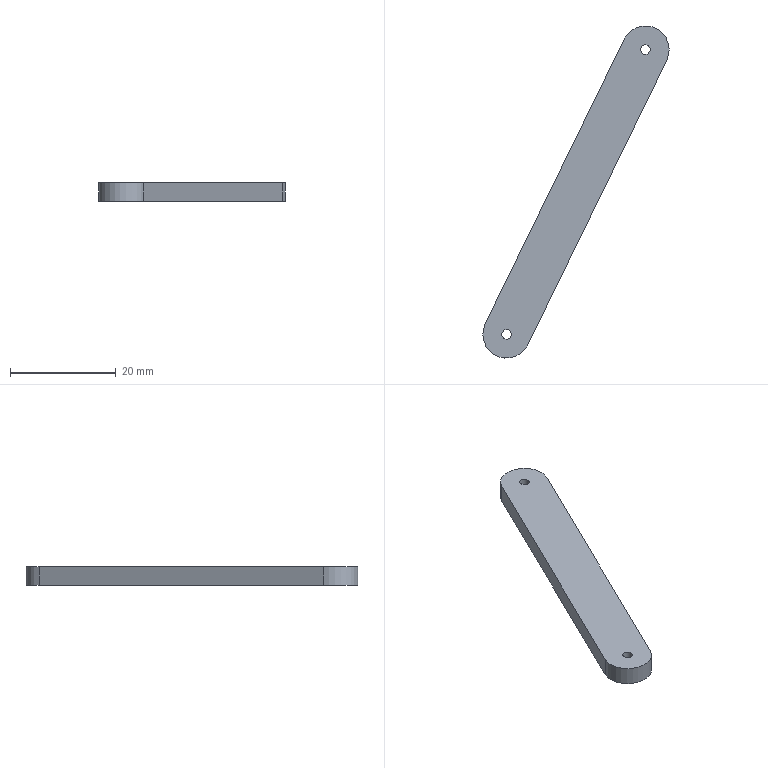Component | NX | SPEAKER_MOUNT | 1 solid | 8 faces | box 35.3 x 62.93 x 3.5 mm | volume 2095 mm3 | cylinder 4 | plane 4 | commonest cylinder face diameters 9 x2 1.8 x2
STEP:
#1=CARTESIAN_POINT('',(0.,0.,0.));
#2=DIRECTION('',(0.,0.,1.));
#3=DIRECTION('',(1.,0.,0.));
#4=AXIS2_PLACEMENT_3D('',#1,#2,#3);
#5=CARTESIAN_POINT('',(33.172,-30.052,31.776));
#6=VERTEX_POINT('',#5);
#7=CARTESIAN_POINT('',(33.172,-30.052,28.276));
#8=VERTEX_POINT('',#7);
#9=CARTESIAN_POINT('',(33.172,-30.052,31.776));
#10=DIRECTION('',(0.,0.,-1.));
#11=VECTOR('',#10,1.);
#12=LINE('',#9,#11);
#13=CARTESIAN_POINT('',(29.127,-28.08,31.776));
#14=DIRECTION('',(0.,0.,-1.));
#15=DIRECTION('',(-1.,0.,0.));
#16=AXIS2_PLACEMENT_3D('',#13,#14,#15);
#17=CYLINDRICAL_SURFACE('',#16,4.5);
#18=CARTESIAN_POINT('',(3.595,0.));
#19=DIRECTION('',(0.,1.));
#20=VECTOR('',#19,1.);
#21=LINE('',#18,#20);
#22=(GEOMETRIC_REPRESENTATION_CONTEXT(2)PARAMETRIC_REPRESENTATION_CONTEXT()REPRESENTATION_CONTEXT('',''));
#23=DEFINITIONAL_REPRESENTATION('',(#21),#22);
#24=PCURVE('',#17,#23);
#25=CARTESIAN_POINT('',(33.172,-30.052,31.776));
#26=DIRECTION('',(-0.8988,0.4384,0.));
#27=DIRECTION('',(-0.4384,-0.8988,0.));
#28=AXIS2_PLACEMENT_3D('',#25,#26,#27);
#29=PLANE('',#28);
#30=CARTESIAN_POINT('',(0.,0.));
#31=DIRECTION('',(0.,-1.));
#32=VECTOR('',#31,1.);
#33=LINE('',#30,#32);
#34=(GEOMETRIC_REPRESENTATION_CONTEXT(2)PARAMETRIC_REPRESENTATION_CONTEXT()REPRESENTATION_CONTEXT('',''));
#35=DEFINITIONAL_REPRESENTATION('',(#33),#34);
#36=PCURVE('',#29,#35);
#37=SURFACE_CURVE('',#12,(#24,#36),.PCURVE_S1.);
#38=EDGE_CURVE('',#6,#8,#37,.T.);
#39=ORIENTED_EDGE('',*,*,#38,.F.);
#40=CARTESIAN_POINT('',(25.083,-26.107,31.776));
#41=VERTEX_POINT('',#40);
#42=CARTESIAN_POINT('',(29.127,-28.08,31.776));
#43=DIRECTION('',(0.,0.,-1.));
#44=DIRECTION('',(1.,0.,0.));
#45=AXIS2_PLACEMENT_3D('',#42,#43,#44);
#46=CIRCLE('',#45,4.5);
#47=CARTESIAN_POINT('',(3.142,0.));
#48=DIRECTION('',(1.,0.));
#49=VECTOR('',#48,1.);
#50=LINE('',#47,#49);
#51=(GEOMETRIC_REPRESENTATION_CONTEXT(2)PARAMETRIC_REPRESENTATION_CONTEXT()REPRESENTATION_CONTEXT('',''));
#52=DEFINITIONAL_REPRESENTATION('',(#50),#51);
#53=PCURVE('',#17,#52);
#54=CARTESIAN_POINT('',(29.127,-28.08,31.776));
#55=DIRECTION('',(0.,0.,1.));
#56=DIRECTION('',(1.,0.,0.));
#57=AXIS2_PLACEMENT_3D('',#54,#55,#56);
#58=PLANE('',#57);
#59=CARTESIAN_POINT('',(4.5,-0.));
#60=CARTESIAN_POINT('',(4.5,-7.794));
#61=CARTESIAN_POINT('',(-2.25,-3.897));
#62=CARTESIAN_POINT('',(-9.,-0.));
#63=CARTESIAN_POINT('',(-2.25,3.897));
#64=CARTESIAN_POINT('',(4.5,7.794));
#65=CARTESIAN_POINT('',(4.5,-0.));
#66=(BOUNDED_CURVE()B_SPLINE_CURVE(2,(#59,#60,#61,#62,#63,#64,#65),.UNSPECIFIED.,.T.,.F.)B_SPLINE_CURVE_WITH_KNOTS((1,2,2,2,2,1),(-2.094,0.,2.094,4.189,6.283,8.378),.UNSPECIFIED.)CURVE()GEOMETRIC_REPRESENTATION_ITEM()RATIONAL_B_SPLINE_CURVE((1.,0.5,1.,0.5,1.,0.5,1.))REPRESENTATION_ITEM(''));
#67=(GEOMETRIC_REPRESENTATION_CONTEXT(2)PARAMETRIC_REPRESENTATION_CONTEXT()REPRESENTATION_CONTEXT('',''));
#68=DEFINITIONAL_REPRESENTATION('',(#66),#67);
#69=PCURVE('',#58,#68);
#70=SURFACE_CURVE('',#46,(#53,#69),.PCURVE_S1.);
#71=EDGE_CURVE('',#6,#41,#70,.T.);
#72=ORIENTED_EDGE('',*,*,#71,.T.);
#73=CARTESIAN_POINT('',(25.083,-26.107,28.276));
#74=VERTEX_POINT('',#73);
#75=CARTESIAN_POINT('',(25.083,-26.107,31.776));
#76=DIRECTION('',(0.,0.,-1.));
#77=VECTOR('',#76,1.);
#78=LINE('',#75,#77);
#79=CARTESIAN_POINT('',(6.737,0.));
#80=DIRECTION('',(0.,1.));
#81=VECTOR('',#80,1.);
#82=LINE('',#79,#81);
#83=(GEOMETRIC_REPRESENTATION_CONTEXT(2)PARAMETRIC_REPRESENTATION_CONTEXT()REPRESENTATION_CONTEXT('',''));
#84=DEFINITIONAL_REPRESENTATION('',(#82),#83);
#85=PCURVE('',#17,#84);
#86=CARTESIAN_POINT('',(51.385,27.821,31.776));
#87=DIRECTION('',(0.8988,-0.4384,0.));
#88=DIRECTION('',(0.4384,0.8988,0.));
#89=AXIS2_PLACEMENT_3D('',#86,#87,#88);
#90=PLANE('',#89);
#91=CARTESIAN_POINT('',(-60.,0.));
#92=DIRECTION('',(0.,-1.));
#93=VECTOR('',#92,1.);
#94=LINE('',#91,#93);
#95=(GEOMETRIC_REPRESENTATION_CONTEXT(2)PARAMETRIC_REPRESENTATION_CONTEXT()REPRESENTATION_CONTEXT('',''));
#96=DEFINITIONAL_REPRESENTATION('',(#94),#95);
#97=PCURVE('',#90,#96);
#98=SURFACE_CURVE('',#78,(#85,#97),.PCURVE_S1.);
#99=EDGE_CURVE('',#41,#74,#98,.T.);
#100=ORIENTED_EDGE('',*,*,#99,.T.);
#101=CARTESIAN_POINT('',(29.127,-28.08,28.276));
#102=DIRECTION('',(0.,0.,-1.));
#103=DIRECTION('',(1.,0.,0.));
#104=AXIS2_PLACEMENT_3D('',#101,#102,#103);
#105=CIRCLE('',#104,4.5);
#106=CARTESIAN_POINT('',(3.142,3.5));
#107=DIRECTION('',(1.,0.));
#108=VECTOR('',#107,1.);
#109=LINE('',#106,#108);
#110=(GEOMETRIC_REPRESENTATION_CONTEXT(2)PARAMETRIC_REPRESENTATION_CONTEXT()REPRESENTATION_CONTEXT('',''));
#111=DEFINITIONAL_REPRESENTATION('',(#109),#110);
#112=PCURVE('',#17,#111);
#113=CARTESIAN_POINT('',(29.127,-28.08,28.276));
#114=DIRECTION('',(0.,0.,1.));
#115=DIRECTION('',(1.,0.,0.));
#116=AXIS2_PLACEMENT_3D('',#113,#114,#115);
#117=PLANE('',#116);
#118=CARTESIAN_POINT('',(4.5,-0.));
#119=CARTESIAN_POINT('',(4.5,-7.794));
#120=CARTESIAN_POINT('',(-2.25,-3.897));
#121=CARTESIAN_POINT('',(-9.,-0.));
#122=CARTESIAN_POINT('',(-2.25,3.897));
#123=CARTESIAN_POINT('',(4.5,7.794));
#124=CARTESIAN_POINT('',(4.5,-0.));
#125=(BOUNDED_CURVE()B_SPLINE_CURVE(2,(#118,#119,#120,#121,#122,#123,#124),.UNSPECIFIED.,.T.,.F.)B_SPLINE_CURVE_WITH_KNOTS((1,2,2,2,2,1),(-2.094,0.,2.094,4.189,6.283,8.378),.UNSPECIFIED.)CURVE()GEOMETRIC_REPRESENTATION_ITEM()RATIONAL_B_SPLINE_CURVE((1.,0.5,1.,0.5,1.,0.5,1.))REPRESENTATION_ITEM(''));
#126=(GEOMETRIC_REPRESENTATION_CONTEXT(2)PARAMETRIC_REPRESENTATION_CONTEXT()REPRESENTATION_CONTEXT('',''));
#127=DEFINITIONAL_REPRESENTATION('',(#125),#126);
#128=PCURVE('',#117,#127);
#129=SURFACE_CURVE('',#105,(#112,#128),.PCURVE_S1.);
#130=EDGE_CURVE('',#8,#74,#129,.T.);
#131=ORIENTED_EDGE('',*,*,#130,.F.);
#132=EDGE_LOOP('',(#39,#72,#100,#131));
#133=FACE_BOUND('',#132,.T.);
#134=ADVANCED_FACE('',(#133),#17,.T.);
#135=CARTESIAN_POINT('',(30.027,-28.08,31.776));
#136=VERTEX_POINT('',#135);
#137=CARTESIAN_POINT('',(29.127,-28.08,31.776));
#138=DIRECTION('',(0.,0.,-1.));
#139=DIRECTION('',(1.,0.,0.));
#140=AXIS2_PLACEMENT_3D('',#137,#138,#139);
#141=CIRCLE('',#140,0.9);
#142=CARTESIAN_POINT('',(29.127,-28.08,31.776));
#143=DIRECTION('',(0.,0.,-1.));
#144=DIRECTION('',(-1.,0.,0.));
#145=AXIS2_PLACEMENT_3D('',#142,#143,#144);
#146=CYLINDRICAL_SURFACE('',#145,0.9);
#147=CARTESIAN_POINT('',(3.142,0.));
#148=DIRECTION('',(1.,0.));
#149=VECTOR('',#148,1.);
#150=LINE('',#147,#149);
#151=(GEOMETRIC_REPRESENTATION_CONTEXT(2)PARAMETRIC_REPRESENTATION_CONTEXT()REPRESENTATION_CONTEXT('',''));
#152=DEFINITIONAL_REPRESENTATION('',(#150),#151);
#153=PCURVE('',#146,#152);
#154=CARTESIAN_POINT('',(0.9,0.));
#155=CARTESIAN_POINT('',(0.9,-1.559));
#156=CARTESIAN_POINT('',(-0.45,-0.7794));
#157=CARTESIAN_POINT('',(-1.8,-0.));
#158=CARTESIAN_POINT('',(-0.45,0.7794));
#159=CARTESIAN_POINT('',(0.9,1.559));
#160=CARTESIAN_POINT('',(0.9,0.));
#161=(BOUNDED_CURVE()B_SPLINE_CURVE(2,(#154,#155,#156,#157,#158,#159,#160),.UNSPECIFIED.,.T.,.F.)B_SPLINE_CURVE_WITH_KNOTS((1,2,2,2,2,1),(-2.094,0.,2.094,4.189,6.283,8.378),.UNSPECIFIED.)CURVE()GEOMETRIC_REPRESENTATION_ITEM()RATIONAL_B_SPLINE_CURVE((1.,0.5,1.,0.5,1.,0.5,1.))REPRESENTATION_ITEM(''));
#162=(GEOMETRIC_REPRESENTATION_CONTEXT(2)PARAMETRIC_REPRESENTATION_CONTEXT()REPRESENTATION_CONTEXT('',''));
#163=DEFINITIONAL_REPRESENTATION('',(#161),#162);
#164=PCURVE('',#58,#163);
#165=SURFACE_CURVE('',#141,(#153,#164),.PCURVE_S1.);
#166=EDGE_CURVE('',#136,#136,#165,.T.);
#167=ORIENTED_EDGE('',*,*,#166,.T.);
#168=CARTESIAN_POINT('',(30.027,-28.08,28.276));
#169=VERTEX_POINT('',#168);
#170=CARTESIAN_POINT('',(30.027,-28.08,31.776));
#171=CARTESIAN_POINT('',(30.027,-28.08,28.276));
#172=B_SPLINE_CURVE_WITH_KNOTS('',1,(#170,#171),.UNSPECIFIED.,.F.,.F.,(2,2),(0.,3.5),.PIECEWISE_BEZIER_KNOTS.);
#173=CARTESIAN_POINT('',(9.425,0.));
#174=DIRECTION('',(0.,1.));
#175=VECTOR('',#174,1.);
#176=LINE('',#173,#175);
#177=(GEOMETRIC_REPRESENTATION_CONTEXT(2)PARAMETRIC_REPRESENTATION_CONTEXT()REPRESENTATION_CONTEXT('',''));
#178=DEFINITIONAL_REPRESENTATION('',(#176),#177);
#179=PCURVE('',#146,#178);
#180=CARTESIAN_POINT('',(3.142,0.));
#181=DIRECTION('',(0.,1.));
#182=VECTOR('',#181,1.);
#183=LINE('',#180,#182);
#184=(GEOMETRIC_REPRESENTATION_CONTEXT(2)PARAMETRIC_REPRESENTATION_CONTEXT()REPRESENTATION_CONTEXT('',''));
#185=DEFINITIONAL_REPRESENTATION('',(#183),#184);
#186=PCURVE('',#146,#185);
#187=SEAM_CURVE('',#172,(#179,#186),.PCURVE_S1.);
#188=EDGE_CURVE('',#136,#169,#187,.T.);
#189=ORIENTED_EDGE('',*,*,#188,.T.);
#190=CARTESIAN_POINT('',(29.127,-28.08,28.276));
#191=DIRECTION('',(0.,0.,-1.));
#192=DIRECTION('',(1.,0.,0.));
#193=AXIS2_PLACEMENT_3D('',#190,#191,#192);
#194=CIRCLE('',#193,0.9);
#195=CARTESIAN_POINT('',(3.142,3.5));
#196=DIRECTION('',(1.,0.));
#197=VECTOR('',#196,1.);
#198=LINE('',#195,#197);
#199=(GEOMETRIC_REPRESENTATION_CONTEXT(2)PARAMETRIC_REPRESENTATION_CONTEXT()REPRESENTATION_CONTEXT('',''));
#200=DEFINITIONAL_REPRESENTATION('',(#198),#199);
#201=PCURVE('',#146,#200);
#202=CARTESIAN_POINT('',(0.9,0.));
#203=CARTESIAN_POINT('',(0.9,-1.559));
#204=CARTESIAN_POINT('',(-0.45,-0.7794));
#205=CARTESIAN_POINT('',(-1.8,-0.));
#206=CARTESIAN_POINT('',(-0.45,0.7794));
#207=CARTESIAN_POINT('',(0.9,1.559));
#208=CARTESIAN_POINT('',(0.9,0.));
#209=(BOUNDED_CURVE()B_SPLINE_CURVE(2,(#202,#203,#204,#205,#206,#207,#208),.UNSPECIFIED.,.T.,.F.)B_SPLINE_CURVE_WITH_KNOTS((1,2,2,2,2,1),(-2.094,0.,2.094,4.189,6.283,8.378),.UNSPECIFIED.)CURVE()GEOMETRIC_REPRESENTATION_ITEM()RATIONAL_B_SPLINE_CURVE((1.,0.5,1.,0.5,1.,0.5,1.))REPRESENTATION_ITEM(''));
#210=(GEOMETRIC_REPRESENTATION_CONTEXT(2)PARAMETRIC_REPRESENTATION_CONTEXT()REPRESENTATION_CONTEXT('',''));
#211=DEFINITIONAL_REPRESENTATION('',(#209),#210);
#212=PCURVE('',#117,#211);
#213=SURFACE_CURVE('',#194,(#201,#212),.PCURVE_S1.);
#214=EDGE_CURVE('',#169,#169,#213,.T.);
#215=ORIENTED_EDGE('',*,*,#214,.F.);
#216=ORIENTED_EDGE('',*,*,#188,.F.);
#217=EDGE_LOOP('',(#167,#189,#215,#216));
#218=FACE_BOUND('',#217,.F.);
#219=ADVANCED_FACE('',(#218),#146,.F.);
#220=ORIENTED_EDGE('',*,*,#71,.F.);
#221=CARTESIAN_POINT('',(59.474,23.875,31.776));
#222=VERTEX_POINT('',#221);
#223=CARTESIAN_POINT('',(33.172,-30.052,31.776));
#224=DIRECTION('',(0.4384,0.8988,0.));
#225=VECTOR('',#224,1.);
#226=LINE('',#223,#225);
#227=CARTESIAN_POINT('',(4.045,-1.973));
#228=DIRECTION('',(0.4384,0.8988));
#229=VECTOR('',#228,1.);
#230=LINE('',#227,#229);
#231=(GEOMETRIC_REPRESENTATION_CONTEXT(2)PARAMETRIC_REPRESENTATION_CONTEXT()REPRESENTATION_CONTEXT('',''));
#232=DEFINITIONAL_REPRESENTATION('',(#230),#231);
#233=PCURVE('',#58,#232);
#234=CARTESIAN_POINT('',(0.,0.));
#235=DIRECTION('',(-1.,0.));
#236=VECTOR('',#235,1.);
#237=LINE('',#234,#236);
#238=(GEOMETRIC_REPRESENTATION_CONTEXT(2)PARAMETRIC_REPRESENTATION_CONTEXT()REPRESENTATION_CONTEXT('',''));
#239=DEFINITIONAL_REPRESENTATION('',(#237),#238);
#240=PCURVE('',#29,#239);
#241=SURFACE_CURVE('',#226,(#233,#240),.PCURVE_S1.);
#242=EDGE_CURVE('',#6,#222,#241,.T.);
#243=ORIENTED_EDGE('',*,*,#242,.T.);
#244=CARTESIAN_POINT('',(51.385,27.821,31.776));
#245=VERTEX_POINT('',#244);
#246=CARTESIAN_POINT('',(55.429,25.848,31.776));
#247=DIRECTION('',(0.,0.,-1.));
#248=DIRECTION('',(1.,0.,0.));
#249=AXIS2_PLACEMENT_3D('',#246,#247,#248);
#250=CIRCLE('',#249,4.5);
#251=CARTESIAN_POINT('',(30.802,53.928));
#252=CARTESIAN_POINT('',(30.802,46.133));
#253=CARTESIAN_POINT('',(24.052,50.031));
#254=CARTESIAN_POINT('',(17.302,53.928));
#255=CARTESIAN_POINT('',(24.052,57.825));
#256=CARTESIAN_POINT('',(30.802,61.722));
#257=CARTESIAN_POINT('',(30.802,53.928));
#258=(BOUNDED_CURVE()B_SPLINE_CURVE(2,(#251,#252,#253,#254,#255,#256,#257),.UNSPECIFIED.,.T.,.F.)B_SPLINE_CURVE_WITH_KNOTS((1,2,2,2,2,1),(-2.094,0.,2.094,4.189,6.283,8.378),.UNSPECIFIED.)CURVE()GEOMETRIC_REPRESENTATION_ITEM()RATIONAL_B_SPLINE_CURVE((1.,0.5,1.,0.5,1.,0.5,1.))REPRESENTATION_ITEM(''));
#259=(GEOMETRIC_REPRESENTATION_CONTEXT(2)PARAMETRIC_REPRESENTATION_CONTEXT()REPRESENTATION_CONTEXT('',''));
#260=DEFINITIONAL_REPRESENTATION('',(#258),#259);
#261=PCURVE('',#58,#260);
#262=CARTESIAN_POINT('',(55.429,25.848,31.776));
#263=DIRECTION('',(0.,0.,-1.));
#264=DIRECTION('',(-1.,0.,0.));
#265=AXIS2_PLACEMENT_3D('',#262,#263,#264);
#266=CYLINDRICAL_SURFACE('',#265,4.5);
#267=CARTESIAN_POINT('',(-3.142,0.));
#268=DIRECTION('',(1.,0.));
#269=VECTOR('',#268,1.);
#270=LINE('',#267,#269);
#271=(GEOMETRIC_REPRESENTATION_CONTEXT(2)PARAMETRIC_REPRESENTATION_CONTEXT()REPRESENTATION_CONTEXT('',''));
#272=DEFINITIONAL_REPRESENTATION('',(#270),#271);
#273=PCURVE('',#266,#272);
#274=SURFACE_CURVE('',#250,(#261,#273),.PCURVE_S1.);
#275=EDGE_CURVE('',#245,#222,#274,.T.);
#276=ORIENTED_EDGE('',*,*,#275,.F.);
#277=CARTESIAN_POINT('',(51.385,27.821,31.776));
#278=DIRECTION('',(-0.4384,-0.8988,0.));
#279=VECTOR('',#278,1.);
#280=LINE('',#277,#279);
#281=CARTESIAN_POINT('',(22.258,55.9));
#282=DIRECTION('',(-0.4384,-0.8988));
#283=VECTOR('',#282,1.);
#284=LINE('',#281,#283);
#285=(GEOMETRIC_REPRESENTATION_CONTEXT(2)PARAMETRIC_REPRESENTATION_CONTEXT()REPRESENTATION_CONTEXT('',''));
#286=DEFINITIONAL_REPRESENTATION('',(#284),#285);
#287=PCURVE('',#58,#286);
#288=CARTESIAN_POINT('',(0.,0.));
#289=DIRECTION('',(-1.,0.));
#290=VECTOR('',#289,1.);
#291=LINE('',#288,#290);
#292=(GEOMETRIC_REPRESENTATION_CONTEXT(2)PARAMETRIC_REPRESENTATION_CONTEXT()REPRESENTATION_CONTEXT('',''));
#293=DEFINITIONAL_REPRESENTATION('',(#291),#292);
#294=PCURVE('',#90,#293);
#295=SURFACE_CURVE('',#280,(#287,#294),.PCURVE_S1.);
#296=EDGE_CURVE('',#245,#41,#295,.T.);
#297=ORIENTED_EDGE('',*,*,#296,.T.);
#298=EDGE_LOOP('',(#220,#243,#276,#297));
#299=FACE_BOUND('',#298,.T.);
#300=ORIENTED_EDGE('',*,*,#166,.T.);
#301=EDGE_LOOP('',(#300));
#302=FACE_BOUND('',#301,.T.);
#303=CARTESIAN_POINT('',(56.329,25.848,31.776));
#304=VERTEX_POINT('',#303);
#305=CARTESIAN_POINT('',(55.429,25.848,31.776));
#306=DIRECTION('',(0.,0.,1.));
#307=DIRECTION('',(1.,0.,0.));
#308=AXIS2_PLACEMENT_3D('',#305,#306,#307);
#309=CIRCLE('',#308,0.9);
#310=CARTESIAN_POINT('',(26.302,53.928));
#311=DIRECTION('',(1.,0.));
#312=AXIS2_PLACEMENT_2D('',#310,#311);
#313=CIRCLE('',#312,0.9);
#314=(GEOMETRIC_REPRESENTATION_CONTEXT(2)PARAMETRIC_REPRESENTATION_CONTEXT()REPRESENTATION_CONTEXT('',''));
#315=DEFINITIONAL_REPRESENTATION('',(#313),#314);
#316=PCURVE('',#58,#315);
#317=CARTESIAN_POINT('',(55.429,25.848,31.776));
#318=DIRECTION('',(0.,0.,-1.));
#319=DIRECTION('',(-1.,0.,0.));
#320=AXIS2_PLACEMENT_3D('',#317,#318,#319);
#321=CYLINDRICAL_SURFACE('',#320,0.9);
#322=CARTESIAN_POINT('',(9.425,0.));
#323=DIRECTION('',(-1.,0.));
#324=VECTOR('',#323,1.);
#325=LINE('',#322,#324);
#326=(GEOMETRIC_REPRESENTATION_CONTEXT(2)PARAMETRIC_REPRESENTATION_CONTEXT()REPRESENTATION_CONTEXT('',''));
#327=DEFINITIONAL_REPRESENTATION('',(#325),#326);
#328=PCURVE('',#321,#327);
#329=SURFACE_CURVE('',#309,(#316,#328),.PCURVE_S1.);
#330=EDGE_CURVE('',#304,#304,#329,.T.);
#331=ORIENTED_EDGE('',*,*,#330,.F.);
#332=EDGE_LOOP('',(#331));
#333=FACE_BOUND('',#332,.T.);
#334=ADVANCED_FACE('',(#299,#302,#333),#58,.T.);
#335=ORIENTED_EDGE('',*,*,#130,.T.);
#336=CARTESIAN_POINT('',(51.385,27.821,28.276));
#337=VERTEX_POINT('',#336);
#338=CARTESIAN_POINT('',(51.385,27.821,28.276));
#339=DIRECTION('',(-0.4384,-0.8988,0.));
#340=VECTOR('',#339,1.);
#341=LINE('',#338,#340);
#342=CARTESIAN_POINT('',(22.258,55.9));
#343=DIRECTION('',(-0.4384,-0.8988));
#344=VECTOR('',#343,1.);
#345=LINE('',#342,#344);
#346=(GEOMETRIC_REPRESENTATION_CONTEXT(2)PARAMETRIC_REPRESENTATION_CONTEXT()REPRESENTATION_CONTEXT('',''));
#347=DEFINITIONAL_REPRESENTATION('',(#345),#346);
#348=PCURVE('',#117,#347);
#349=CARTESIAN_POINT('',(0.,-3.5));
#350=DIRECTION('',(-1.,0.));
#351=VECTOR('',#350,1.);
#352=LINE('',#349,#351);
#353=(GEOMETRIC_REPRESENTATION_CONTEXT(2)PARAMETRIC_REPRESENTATION_CONTEXT()REPRESENTATION_CONTEXT('',''));
#354=DEFINITIONAL_REPRESENTATION('',(#352),#353);
#355=PCURVE('',#90,#354);
#356=SURFACE_CURVE('',#341,(#348,#355),.PCURVE_S1.);
#357=EDGE_CURVE('',#337,#74,#356,.T.);
#358=ORIENTED_EDGE('',*,*,#357,.F.);
#359=CARTESIAN_POINT('',(59.474,23.875,28.276));
#360=VERTEX_POINT('',#359);
#361=CARTESIAN_POINT('',(55.429,25.848,28.276));
#362=DIRECTION('',(0.,0.,-1.));
#363=DIRECTION('',(1.,0.,0.));
#364=AXIS2_PLACEMENT_3D('',#361,#362,#363);
#365=CIRCLE('',#364,4.5);
#366=CARTESIAN_POINT('',(30.802,53.928));
#367=CARTESIAN_POINT('',(30.802,46.133));
#368=CARTESIAN_POINT('',(24.052,50.031));
#369=CARTESIAN_POINT('',(17.302,53.928));
#370=CARTESIAN_POINT('',(24.052,57.825));
#371=CARTESIAN_POINT('',(30.802,61.722));
#372=CARTESIAN_POINT('',(30.802,53.928));
#373=(BOUNDED_CURVE()B_SPLINE_CURVE(2,(#366,#367,#368,#369,#370,#371,#372),.UNSPECIFIED.,.T.,.F.)B_SPLINE_CURVE_WITH_KNOTS((1,2,2,2,2,1),(-2.094,0.,2.094,4.189,6.283,8.378),.UNSPECIFIED.)CURVE()GEOMETRIC_REPRESENTATION_ITEM()RATIONAL_B_SPLINE_CURVE((1.,0.5,1.,0.5,1.,0.5,1.))REPRESENTATION_ITEM(''));
#374=(GEOMETRIC_REPRESENTATION_CONTEXT(2)PARAMETRIC_REPRESENTATION_CONTEXT()REPRESENTATION_CONTEXT('',''));
#375=DEFINITIONAL_REPRESENTATION('',(#373),#374);
#376=PCURVE('',#117,#375);
#377=CARTESIAN_POINT('',(-3.142,3.5));
#378=DIRECTION('',(1.,0.));
#379=VECTOR('',#378,1.);
#380=LINE('',#377,#379);
#381=(GEOMETRIC_REPRESENTATION_CONTEXT(2)PARAMETRIC_REPRESENTATION_CONTEXT()REPRESENTATION_CONTEXT('',''));
#382=DEFINITIONAL_REPRESENTATION('',(#380),#381);
#383=PCURVE('',#266,#382);
#384=SURFACE_CURVE('',#365,(#376,#383),.PCURVE_S1.);
#385=EDGE_CURVE('',#337,#360,#384,.T.);
#386=ORIENTED_EDGE('',*,*,#385,.T.);
#387=CARTESIAN_POINT('',(33.172,-30.052,28.276));
#388=DIRECTION('',(0.4384,0.8988,0.));
#389=VECTOR('',#388,1.);
#390=LINE('',#387,#389);
#391=CARTESIAN_POINT('',(4.045,-1.973));
#392=DIRECTION('',(0.4384,0.8988));
#393=VECTOR('',#392,1.);
#394=LINE('',#391,#393);
#395=(GEOMETRIC_REPRESENTATION_CONTEXT(2)PARAMETRIC_REPRESENTATION_CONTEXT()REPRESENTATION_CONTEXT('',''));
#396=DEFINITIONAL_REPRESENTATION('',(#394),#395);
#397=PCURVE('',#117,#396);
#398=CARTESIAN_POINT('',(0.,-3.5));
#399=DIRECTION('',(-1.,0.));
#400=VECTOR('',#399,1.);
#401=LINE('',#398,#400);
#402=(GEOMETRIC_REPRESENTATION_CONTEXT(2)PARAMETRIC_REPRESENTATION_CONTEXT()REPRESENTATION_CONTEXT('',''));
#403=DEFINITIONAL_REPRESENTATION('',(#401),#402);
#404=PCURVE('',#29,#403);
#405=SURFACE_CURVE('',#390,(#397,#404),.PCURVE_S1.);
#406=EDGE_CURVE('',#8,#360,#405,.T.);
#407=ORIENTED_EDGE('',*,*,#406,.F.);
#408=EDGE_LOOP('',(#335,#358,#386,#407));
#409=FACE_BOUND('',#408,.T.);
#410=ORIENTED_EDGE('',*,*,#214,.F.);
#411=EDGE_LOOP('',(#410));
#412=FACE_BOUND('',#411,.T.);
#413=CARTESIAN_POINT('',(56.329,25.848,28.276));
#414=VERTEX_POINT('',#413);
#415=CARTESIAN_POINT('',(55.429,25.848,28.276));
#416=DIRECTION('',(0.,0.,1.));
#417=DIRECTION('',(1.,0.,0.));
#418=AXIS2_PLACEMENT_3D('',#415,#416,#417);
#419=CIRCLE('',#418,0.9);
#420=CARTESIAN_POINT('',(26.302,53.928));
#421=DIRECTION('',(1.,0.));
#422=AXIS2_PLACEMENT_2D('',#420,#421);
#423=CIRCLE('',#422,0.9);
#424=(GEOMETRIC_REPRESENTATION_CONTEXT(2)PARAMETRIC_REPRESENTATION_CONTEXT()REPRESENTATION_CONTEXT('',''));
#425=DEFINITIONAL_REPRESENTATION('',(#423),#424);
#426=PCURVE('',#117,#425);
#427=CARTESIAN_POINT('',(9.425,3.5));
#428=DIRECTION('',(-1.,0.));
#429=VECTOR('',#428,1.);
#430=LINE('',#427,#429);
#431=(GEOMETRIC_REPRESENTATION_CONTEXT(2)PARAMETRIC_REPRESENTATION_CONTEXT()REPRESENTATION_CONTEXT('',''));
#432=DEFINITIONAL_REPRESENTATION('',(#430),#431);
#433=PCURVE('',#321,#432);
#434=SURFACE_CURVE('',#419,(#426,#433),.PCURVE_S1.);
#435=EDGE_CURVE('',#414,#414,#434,.T.);
#436=ORIENTED_EDGE('',*,*,#435,.T.);
#437=EDGE_LOOP('',(#436));
#438=FACE_BOUND('',#437,.T.);
#439=ADVANCED_FACE('',(#409,#412,#438),#117,.F.);
#440=ORIENTED_EDGE('',*,*,#406,.T.);
#441=CARTESIAN_POINT('',(59.474,23.875,31.776));
#442=DIRECTION('',(0.,0.,-1.));
#443=VECTOR('',#442,1.);
#444=LINE('',#441,#443);
#445=CARTESIAN_POINT('',(-60.,0.));
#446=DIRECTION('',(0.,-1.));
#447=VECTOR('',#446,1.);
#448=LINE('',#445,#447);
#449=(GEOMETRIC_REPRESENTATION_CONTEXT(2)PARAMETRIC_REPRESENTATION_CONTEXT()REPRESENTATION_CONTEXT('',''));
#450=DEFINITIONAL_REPRESENTATION('',(#448),#449);
#451=PCURVE('',#29,#450);
#452=CARTESIAN_POINT('',(3.595,0.));
#453=DIRECTION('',(0.,1.));
#454=VECTOR('',#453,1.);
#455=LINE('',#452,#454);
#456=(GEOMETRIC_REPRESENTATION_CONTEXT(2)PARAMETRIC_REPRESENTATION_CONTEXT()REPRESENTATION_CONTEXT('',''));
#457=DEFINITIONAL_REPRESENTATION('',(#455),#456);
#458=PCURVE('',#266,#457);
#459=SURFACE_CURVE('',#444,(#451,#458),.PCURVE_S1.);
#460=EDGE_CURVE('',#222,#360,#459,.T.);
#461=ORIENTED_EDGE('',*,*,#460,.F.);
#462=ORIENTED_EDGE('',*,*,#242,.F.);
#463=ORIENTED_EDGE('',*,*,#38,.T.);
#464=EDGE_LOOP('',(#440,#461,#462,#463));
#465=FACE_BOUND('',#464,.T.);
#466=ADVANCED_FACE('',(#465),#29,.F.);
#467=ORIENTED_EDGE('',*,*,#357,.T.);
#468=ORIENTED_EDGE('',*,*,#99,.F.);
#469=ORIENTED_EDGE('',*,*,#296,.F.);
#470=CARTESIAN_POINT('',(51.385,27.821,31.776));
#471=DIRECTION('',(0.,0.,-1.));
#472=VECTOR('',#471,1.);
#473=LINE('',#470,#472);
#474=CARTESIAN_POINT('',(0.,0.));
#475=DIRECTION('',(0.,-1.));
#476=VECTOR('',#475,1.);
#477=LINE('',#474,#476);
#478=(GEOMETRIC_REPRESENTATION_CONTEXT(2)PARAMETRIC_REPRESENTATION_CONTEXT()REPRESENTATION_CONTEXT('',''));
#479=DEFINITIONAL_REPRESENTATION('',(#477),#478);
#480=PCURVE('',#90,#479);
#481=CARTESIAN_POINT('',(0.4538,0.));
#482=DIRECTION('',(0.,1.));
#483=VECTOR('',#482,1.);
#484=LINE('',#481,#483);
#485=(GEOMETRIC_REPRESENTATION_CONTEXT(2)PARAMETRIC_REPRESENTATION_CONTEXT()REPRESENTATION_CONTEXT('',''));
#486=DEFINITIONAL_REPRESENTATION('',(#484),#485);
#487=PCURVE('',#266,#486);
#488=SURFACE_CURVE('',#473,(#480,#487),.PCURVE_S1.);
#489=EDGE_CURVE('',#245,#337,#488,.T.);
#490=ORIENTED_EDGE('',*,*,#489,.T.);
#491=EDGE_LOOP('',(#467,#468,#469,#490));
#492=FACE_BOUND('',#491,.T.);
#493=ADVANCED_FACE('',(#492),#90,.F.);
#494=ORIENTED_EDGE('',*,*,#489,.F.);
#495=ORIENTED_EDGE('',*,*,#275,.T.);
#496=ORIENTED_EDGE('',*,*,#460,.T.);
#497=ORIENTED_EDGE('',*,*,#385,.F.);
#498=EDGE_LOOP('',(#494,#495,#496,#497));
#499=FACE_BOUND('',#498,.T.);
#500=ADVANCED_FACE('',(#499),#266,.T.);
#501=ORIENTED_EDGE('',*,*,#330,.F.);
#502=CARTESIAN_POINT('',(56.329,25.848,31.776));
#503=CARTESIAN_POINT('',(56.329,25.848,28.276));
#504=B_SPLINE_CURVE_WITH_KNOTS('',1,(#502,#503),.UNSPECIFIED.,.F.,.F.,(2,2),(0.,3.5),.PIECEWISE_BEZIER_KNOTS.);
#505=CARTESIAN_POINT('',(9.425,0.));
#506=DIRECTION('',(0.,1.));
#507=VECTOR('',#506,1.);
#508=LINE('',#505,#507);
#509=(GEOMETRIC_REPRESENTATION_CONTEXT(2)PARAMETRIC_REPRESENTATION_CONTEXT()REPRESENTATION_CONTEXT('',''));
#510=DEFINITIONAL_REPRESENTATION('',(#508),#509);
#511=PCURVE('',#321,#510);
#512=CARTESIAN_POINT('',(3.142,0.));
#513=DIRECTION('',(0.,1.));
#514=VECTOR('',#513,1.);
#515=LINE('',#512,#514);
#516=(GEOMETRIC_REPRESENTATION_CONTEXT(2)PARAMETRIC_REPRESENTATION_CONTEXT()REPRESENTATION_CONTEXT('',''));
#517=DEFINITIONAL_REPRESENTATION('',(#515),#516);
#518=PCURVE('',#321,#517);
#519=SEAM_CURVE('',#504,(#511,#518),.PCURVE_S1.);
#520=EDGE_CURVE('',#304,#414,#519,.T.);
#521=ORIENTED_EDGE('',*,*,#520,.T.);
#522=ORIENTED_EDGE('',*,*,#435,.T.);
#523=ORIENTED_EDGE('',*,*,#520,.F.);
#524=EDGE_LOOP('',(#501,#521,#522,#523));
#525=FACE_BOUND('',#524,.F.);
#526=ADVANCED_FACE('',(#525),#321,.F.);
#527=CLOSED_SHELL('',(#134,#219,#334,#439,#466,#493,#500,#526));
#528=MANIFOLD_SOLID_BREP('',#527);
#529=(LENGTH_UNIT()NAMED_UNIT(*)SI_UNIT(.MILLI.,.METRE.));
#530=UNCERTAINTY_MEASURE_WITH_UNIT(LENGTH_MEASURE(0.000002),#529,'','');
#531=(NAMED_UNIT(*)PLANE_ANGLE_UNIT()SI_UNIT($,.RADIAN.));
#532=(NAMED_UNIT(*)SI_UNIT($,.STERADIAN.)SOLID_ANGLE_UNIT());
#533=(GEOMETRIC_REPRESENTATION_CONTEXT(3)GLOBAL_UNCERTAINTY_ASSIGNED_CONTEXT((#530))GLOBAL_UNIT_ASSIGNED_CONTEXT((#529,#531,#532))REPRESENTATION_CONTEXT('',''));
#534=ADVANCED_BREP_SHAPE_REPRESENTATION('',(#4,#528),#533);